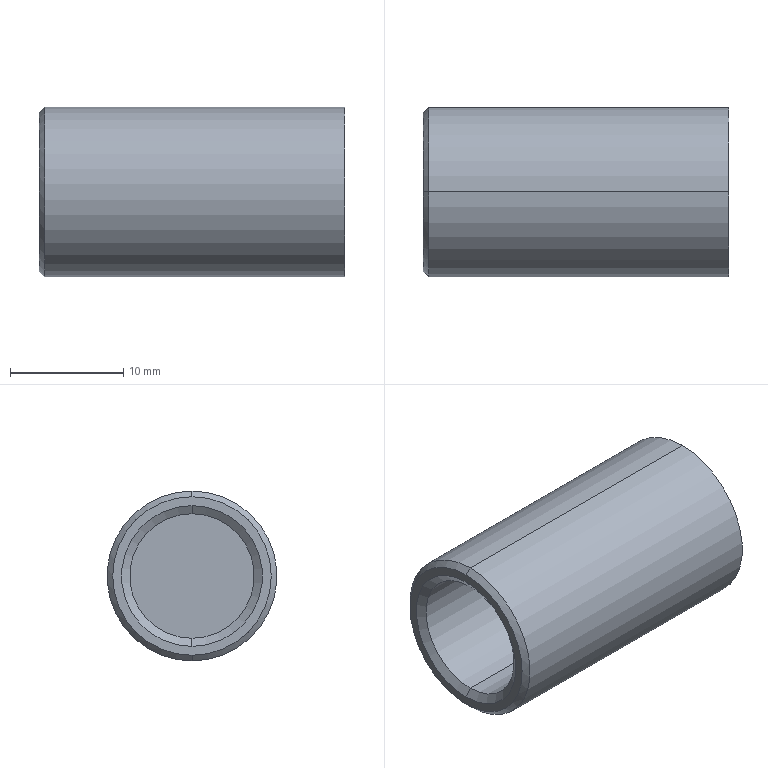Component | SolidWorks | LocatingPin-1 | 1 solid | 11 faces | box 27 x 15 x 15 mm | volume 2953 mm3 | cylinder 4 | cone 4 | plane 3 | commonest cylinder face diameters 11 x2 15 x2 | material Alloy Steel
build123d program:
from build123d import *


with BuildPart() as part:
    # Model → Revolve1 (revolve)
    with BuildSketch(Plane.XY, mode=Mode.PRIVATE) as revolve1_sk:
        Polygon((10.636, 8.083), (-15.864, 8.083), (-16.364, 7.583), (-16.364, 6.802), (-15.864, 6.083), (2.636, 6.083), (2.636, 0.5825), (10.636, 0.5825), align=None)
    revolve(revolve1_sk.sketch.rotate(Axis((10.636, 0.5825, 0), (-1, 0, 0)), 90), axis=Axis((10.636, 0.5825, 0), (-1, 0, 0)))


solid = part.part

# Placed as in the assembly
solid = solid.moved(Location((92.868, -0.6058, -0.0004174), (0, 0, 0)))
STEP:
#1=COLOUR_RGB('',0.7922,0.8196,0.9333);
#2=FILL_AREA_STYLE_COLOUR('',#1);
#3=FILL_AREA_STYLE('',(#2));
#4=SURFACE_STYLE_FILL_AREA(#3);
#5=SURFACE_SIDE_STYLE('',(#4));
#6=SURFACE_STYLE_USAGE(.BOTH.,#5);
#7=PRESENTATION_STYLE_ASSIGNMENT((#6));
#8=CARTESIAN_POINT('',(3.032,-0.0009151,0.2165));
#9=VERTEX_POINT('',#8);
#10=CARTESIAN_POINT('',(3.032,-0.0009151,-0.2166));
#11=VERTEX_POINT('',#10);
#12=CARTESIAN_POINT('',(3.032,-0.0009151,-0.00001643));
#13=DIRECTION('',(1.,0.,0.));
#14=DIRECTION('',(0.,0.,-1.));
#15=AXIS2_PLACEMENT_3D('',#12,#13,#14);
#16=CIRCLE('',#15,0.2165);
#17=EDGE_CURVE('',#9,#11,#16,.T.);
#18=ORIENTED_EDGE('',*,*,#17,.F.);
#19=CARTESIAN_POINT('',(3.76,-0.0009151,0.2165));
#20=VERTEX_POINT('',#19);
#21=CARTESIAN_POINT('',(4.075,-0.0009151,0.2165));
#22=DIRECTION('',(1.,0.,0.));
#23=VECTOR('',#22,39.37);
#24=LINE('',#21,#23);
#25=EDGE_CURVE('',#9,#20,#24,.T.);
#26=ORIENTED_EDGE('',*,*,#25,.T.);
#27=CARTESIAN_POINT('',(3.76,-0.0009151,-0.2166));
#28=VERTEX_POINT('',#27);
#29=CARTESIAN_POINT('',(3.76,-0.0009151,-0.00001643));
#30=DIRECTION('',(1.,0.,0.));
#31=DIRECTION('',(0.,0.,-1.));
#32=AXIS2_PLACEMENT_3D('',#29,#30,#31);
#33=CIRCLE('',#32,0.2165);
#34=EDGE_CURVE('',#20,#28,#33,.T.);
#35=ORIENTED_EDGE('',*,*,#34,.T.);
#36=CARTESIAN_POINT('',(4.075,-0.0009151,-0.2166));
#37=DIRECTION('',(1.,0.,0.));
#38=VECTOR('',#37,39.37);
#39=LINE('',#36,#38);
#40=EDGE_CURVE('',#11,#28,#39,.T.);
#41=ORIENTED_EDGE('',*,*,#40,.F.);
#42=EDGE_LOOP('',(#18,#26,#35,#41));
#43=FACE_OUTER_BOUND('',#42,.T.);
#44=CARTESIAN_POINT('',(4.075,-0.0009151,-0.00001643));
#45=DIRECTION('',(1.,0.,0.));
#46=DIRECTION('',(0.,0.,-1.));
#47=AXIS2_PLACEMENT_3D('',#44,#45,#46);
#48=CYLINDRICAL_SURFACE('',#47,0.2165);
#49=ADVANCED_FACE('',(#43),#48,.F.);
#50=ORIENTED_EDGE('',*,*,#17,.T.);
#51=CARTESIAN_POINT('',(3.012,-0.0009151,-0.2449));
#52=VERTEX_POINT('',#51);
#53=CARTESIAN_POINT('',(3.012,-0.0009151,-0.2449));
#54=DIRECTION('',(-0.5705,0.,-0.8213));
#55=VECTOR('',#54,39.37);
#56=LINE('',#53,#55);
#57=EDGE_CURVE('',#11,#52,#56,.T.);
#58=ORIENTED_EDGE('',*,*,#57,.T.);
#59=CARTESIAN_POINT('',(3.012,-0.0009151,0.2449));
#60=VERTEX_POINT('',#59);
#61=CARTESIAN_POINT('',(3.012,-0.0009151,-0.00001643));
#62=DIRECTION('',(1.,0.,0.));
#63=DIRECTION('',(0.,0.,-1.));
#64=AXIS2_PLACEMENT_3D('',#61,#62,#63);
#65=CIRCLE('',#64,0.2449);
#66=EDGE_CURVE('',#60,#52,#65,.T.);
#67=ORIENTED_EDGE('',*,*,#66,.F.);
#68=CARTESIAN_POINT('',(3.012,-0.0009151,0.2449));
#69=DIRECTION('',(-0.5705,0.,0.8213));
#70=VECTOR('',#69,39.37);
#71=LINE('',#68,#70);
#72=EDGE_CURVE('',#9,#60,#71,.T.);
#73=ORIENTED_EDGE('',*,*,#72,.F.);
#74=EDGE_LOOP('',(#50,#58,#67,#73));
#75=FACE_OUTER_BOUND('',#74,.T.);
#76=CARTESIAN_POINT('',(3.012,-0.0009151,-0.00001643));
#77=DIRECTION('',(-1.,0.,0.));
#78=DIRECTION('',(0.,0.,1.));
#79=AXIS2_PLACEMENT_3D('',#76,#77,#78);
#80=CONICAL_SURFACE('',#79,0.2449,0.9637);
#81=ADVANCED_FACE('',(#75),#80,.F.);
#82=CARTESIAN_POINT('',(3.012,-0.0009151,-0.2756));
#83=VERTEX_POINT('',#82);
#84=CARTESIAN_POINT('',(3.012,-0.0009151,0.2756));
#85=VERTEX_POINT('',#84);
#86=CARTESIAN_POINT('',(3.012,-0.0009151,-0.00001643));
#87=DIRECTION('',(1.,0.,0.));
#88=DIRECTION('',(0.,0.,-1.));
#89=AXIS2_PLACEMENT_3D('',#86,#87,#88);
#90=CIRCLE('',#89,0.2756);
#91=EDGE_CURVE('',#83,#85,#90,.T.);
#92=ORIENTED_EDGE('',*,*,#91,.T.);
#93=CARTESIAN_POINT('',(3.032,-0.0009151,0.2953));
#94=VERTEX_POINT('',#93);
#95=CARTESIAN_POINT('',(3.032,-0.0009151,0.2953));
#96=DIRECTION('',(0.7071,0.,0.7071));
#97=VECTOR('',#96,39.37);
#98=LINE('',#95,#97);
#99=EDGE_CURVE('',#85,#94,#98,.T.);
#100=ORIENTED_EDGE('',*,*,#99,.T.);
#101=CARTESIAN_POINT('',(3.032,-0.0009151,-0.2953));
#102=VERTEX_POINT('',#101);
#103=CARTESIAN_POINT('',(3.032,-0.0009151,-0.00001643));
#104=DIRECTION('',(1.,0.,0.));
#105=DIRECTION('',(0.,0.,-1.));
#106=AXIS2_PLACEMENT_3D('',#103,#104,#105);
#107=CIRCLE('',#106,0.2953);
#108=EDGE_CURVE('',#102,#94,#107,.T.);
#109=ORIENTED_EDGE('',*,*,#108,.F.);
#110=CARTESIAN_POINT('',(3.032,-0.0009151,-0.2953));
#111=DIRECTION('',(0.7071,0.,-0.7071));
#112=VECTOR('',#111,39.37);
#113=LINE('',#110,#112);
#114=EDGE_CURVE('',#83,#102,#113,.T.);
#115=ORIENTED_EDGE('',*,*,#114,.F.);
#116=EDGE_LOOP('',(#92,#100,#109,#115));
#117=FACE_OUTER_BOUND('',#116,.T.);
#118=CARTESIAN_POINT('',(3.032,-0.0009151,-0.00001643));
#119=DIRECTION('',(1.,0.,0.));
#120=DIRECTION('',(0.,0.,-1.));
#121=AXIS2_PLACEMENT_3D('',#118,#119,#120);
#122=CONICAL_SURFACE('',#121,0.2953,0.7854);
#123=ADVANCED_FACE('',(#117),#122,.T.);
#124=ORIENTED_EDGE('',*,*,#108,.T.);
#125=CARTESIAN_POINT('',(4.075,-0.0009151,0.2953));
#126=VERTEX_POINT('',#125);
#127=CARTESIAN_POINT('',(4.075,-0.0009151,0.2953));
#128=DIRECTION('',(1.,0.,0.));
#129=VECTOR('',#128,39.37);
#130=LINE('',#127,#129);
#131=EDGE_CURVE('',#94,#126,#130,.T.);
#132=ORIENTED_EDGE('',*,*,#131,.T.);
#133=CARTESIAN_POINT('',(4.075,-0.0009151,-0.2953));
#134=VERTEX_POINT('',#133);
#135=CARTESIAN_POINT('',(4.075,-0.0009151,-0.00001643));
#136=DIRECTION('',(1.,0.,0.));
#137=DIRECTION('',(0.,0.,-1.));
#138=AXIS2_PLACEMENT_3D('',#135,#136,#137);
#139=CIRCLE('',#138,0.2953);
#140=EDGE_CURVE('',#134,#126,#139,.T.);
#141=ORIENTED_EDGE('',*,*,#140,.F.);
#142=CARTESIAN_POINT('',(4.075,-0.0009151,-0.2953));
#143=DIRECTION('',(1.,0.,0.));
#144=VECTOR('',#143,39.37);
#145=LINE('',#142,#144);
#146=EDGE_CURVE('',#102,#134,#145,.T.);
#147=ORIENTED_EDGE('',*,*,#146,.F.);
#148=EDGE_LOOP('',(#124,#132,#141,#147));
#149=FACE_OUTER_BOUND('',#148,.T.);
#150=CARTESIAN_POINT('',(4.075,-0.0009151,-0.00001643));
#151=DIRECTION('',(1.,0.,0.));
#152=DIRECTION('',(0.,0.,-1.));
#153=AXIS2_PLACEMENT_3D('',#150,#151,#152);
#154=CYLINDRICAL_SURFACE('',#153,0.2953);
#155=ADVANCED_FACE('',(#149),#154,.T.);
#156=ORIENTED_EDGE('',*,*,#140,.T.);
#157=CARTESIAN_POINT('',(4.075,-0.0009151,-0.00001643));
#158=DIRECTION('',(1.,0.,0.));
#159=DIRECTION('',(0.,0.,-1.));
#160=AXIS2_PLACEMENT_3D('',#157,#158,#159);
#161=CIRCLE('',#160,0.2953);
#162=EDGE_CURVE('',#126,#134,#161,.T.);
#163=ORIENTED_EDGE('',*,*,#162,.T.);
#164=EDGE_LOOP('',(#156,#163));
#165=FACE_OUTER_BOUND('',#164,.T.);
#166=CARTESIAN_POINT('',(4.075,-0.0009151,-0.00001643));
#167=DIRECTION('',(1.,0.,0.));
#168=DIRECTION('',(0.,0.,-1.));
#169=AXIS2_PLACEMENT_3D('',#166,#167,#168);
#170=PLANE('',#169);
#171=ADVANCED_FACE('',(#165),#170,.T.);
#172=ORIENTED_EDGE('',*,*,#131,.F.);
#173=CARTESIAN_POINT('',(3.032,-0.0009151,-0.00001643));
#174=DIRECTION('',(1.,0.,0.));
#175=DIRECTION('',(0.,0.,-1.));
#176=AXIS2_PLACEMENT_3D('',#173,#174,#175);
#177=CIRCLE('',#176,0.2953);
#178=EDGE_CURVE('',#94,#102,#177,.T.);
#179=ORIENTED_EDGE('',*,*,#178,.T.);
#180=ORIENTED_EDGE('',*,*,#146,.T.);
#181=ORIENTED_EDGE('',*,*,#162,.F.);
#182=EDGE_LOOP('',(#172,#179,#180,#181));
#183=FACE_OUTER_BOUND('',#182,.T.);
#184=CARTESIAN_POINT('',(4.075,-0.0009151,-0.00001643));
#185=DIRECTION('',(1.,0.,0.));
#186=DIRECTION('',(0.,0.,-1.));
#187=AXIS2_PLACEMENT_3D('',#184,#185,#186);
#188=CYLINDRICAL_SURFACE('',#187,0.2953);
#189=ADVANCED_FACE('',(#183),#188,.T.);
#190=ORIENTED_EDGE('',*,*,#99,.F.);
#191=CARTESIAN_POINT('',(3.012,-0.0009151,-0.00001643));
#192=DIRECTION('',(1.,0.,0.));
#193=DIRECTION('',(0.,0.,-1.));
#194=AXIS2_PLACEMENT_3D('',#191,#192,#193);
#195=CIRCLE('',#194,0.2756);
#196=EDGE_CURVE('',#85,#83,#195,.T.);
#197=ORIENTED_EDGE('',*,*,#196,.T.);
#198=ORIENTED_EDGE('',*,*,#114,.T.);
#199=ORIENTED_EDGE('',*,*,#178,.F.);
#200=EDGE_LOOP('',(#190,#197,#198,#199));
#201=FACE_OUTER_BOUND('',#200,.T.);
#202=CARTESIAN_POINT('',(3.032,-0.0009151,-0.00001643));
#203=DIRECTION('',(1.,0.,0.));
#204=DIRECTION('',(0.,0.,-1.));
#205=AXIS2_PLACEMENT_3D('',#202,#203,#204);
#206=CONICAL_SURFACE('',#205,0.2953,0.7854);
#207=ADVANCED_FACE('',(#201),#206,.T.);
#208=ORIENTED_EDGE('',*,*,#66,.T.);
#209=CARTESIAN_POINT('',(3.012,-0.0009151,-0.00001643));
#210=DIRECTION('',(1.,0.,0.));
#211=DIRECTION('',(0.,0.,-1.));
#212=AXIS2_PLACEMENT_3D('',#209,#210,#211);
#213=CIRCLE('',#212,0.2449);
#214=EDGE_CURVE('',#52,#60,#213,.T.);
#215=ORIENTED_EDGE('',*,*,#214,.T.);
#216=EDGE_LOOP('',(#208,#215));
#217=FACE_BOUND('',#216,.T.);
#218=ORIENTED_EDGE('',*,*,#91,.F.);
#219=ORIENTED_EDGE('',*,*,#196,.F.);
#220=EDGE_LOOP('',(#218,#219));
#221=FACE_OUTER_BOUND('',#220,.T.);
#222=CARTESIAN_POINT('',(3.012,0.244,-0.00001643));
#223=DIRECTION('',(-1.,0.,0.));
#224=DIRECTION('',(0.,0.,1.));
#225=AXIS2_PLACEMENT_3D('',#222,#223,#224);
#226=PLANE('',#225);
#227=ADVANCED_FACE('',(#217,#221),#226,.T.);
#228=ORIENTED_EDGE('',*,*,#57,.F.);
#229=CARTESIAN_POINT('',(3.032,-0.0009151,-0.00001643));
#230=DIRECTION('',(1.,0.,0.));
#231=DIRECTION('',(0.,0.,-1.));
#232=AXIS2_PLACEMENT_3D('',#229,#230,#231);
#233=CIRCLE('',#232,0.2165);
#234=EDGE_CURVE('',#11,#9,#233,.T.);
#235=ORIENTED_EDGE('',*,*,#234,.T.);
#236=ORIENTED_EDGE('',*,*,#72,.T.);
#237=ORIENTED_EDGE('',*,*,#214,.F.);
#238=EDGE_LOOP('',(#228,#235,#236,#237));
#239=FACE_OUTER_BOUND('',#238,.T.);
#240=CARTESIAN_POINT('',(3.012,-0.0009151,-0.00001643));
#241=DIRECTION('',(-1.,0.,0.));
#242=DIRECTION('',(0.,0.,1.));
#243=AXIS2_PLACEMENT_3D('',#240,#241,#242);
#244=CONICAL_SURFACE('',#243,0.2449,0.9637);
#245=ADVANCED_FACE('',(#239),#244,.F.);
#246=ORIENTED_EDGE('',*,*,#25,.F.);
#247=ORIENTED_EDGE('',*,*,#234,.F.);
#248=ORIENTED_EDGE('',*,*,#40,.T.);
#249=CARTESIAN_POINT('',(3.76,-0.0009151,-0.00001643));
#250=DIRECTION('',(1.,0.,0.));
#251=DIRECTION('',(0.,0.,-1.));
#252=AXIS2_PLACEMENT_3D('',#249,#250,#251);
#253=CIRCLE('',#252,0.2165);
#254=EDGE_CURVE('',#28,#20,#253,.T.);
#255=ORIENTED_EDGE('',*,*,#254,.T.);
#256=EDGE_LOOP('',(#246,#247,#248,#255));
#257=FACE_OUTER_BOUND('',#256,.T.);
#258=CARTESIAN_POINT('',(4.075,-0.0009151,-0.00001643));
#259=DIRECTION('',(1.,0.,0.));
#260=DIRECTION('',(0.,0.,-1.));
#261=AXIS2_PLACEMENT_3D('',#258,#259,#260);
#262=CYLINDRICAL_SURFACE('',#261,0.2165);
#263=ADVANCED_FACE('',(#257),#262,.F.);
#264=ORIENTED_EDGE('',*,*,#254,.F.);
#265=ORIENTED_EDGE('',*,*,#34,.F.);
#266=EDGE_LOOP('',(#264,#265));
#267=FACE_OUTER_BOUND('',#266,.T.);
#268=CARTESIAN_POINT('',(3.76,-0.0009151,-0.00001643));
#269=DIRECTION('',(-1.,0.,0.));
#270=DIRECTION('',(0.,0.,1.));
#271=AXIS2_PLACEMENT_3D('',#268,#269,#270);
#272=PLANE('',#271);
#273=ADVANCED_FACE('',(#267),#272,.T.);
#274=CLOSED_SHELL('',(#49,#81,#123,#155,#171,#189,#207,#227,#245,#263,#273));
#275=MANIFOLD_SOLID_BREP('',#274);
#276=STYLED_ITEM('',(#7),#275);
#277=PRESENTATION_LAYER_ASSIGNMENT('','',(#276));
#278=CARTESIAN_POINT('',(0.,0.,0.));
#279=DIRECTION('',(0.,0.,1.));
#280=DIRECTION('',(1.,0.,0.));
#281=AXIS2_PLACEMENT_3D('',#278,#279,#280);
#282=(LENGTH_UNIT()NAMED_UNIT(*)SI_UNIT($,.METRE.));
#283=LENGTH_MEASURE_WITH_UNIT(LENGTH_MEASURE(0.0254),#282);
#284=DIMENSIONAL_EXPONENTS(1.,0.,0.,0.,0.,0.,0.);
#285=(CONVERSION_BASED_UNIT('',#283)LENGTH_UNIT()NAMED_UNIT(#284));
#286=UNCERTAINTY_MEASURE_WITH_UNIT(LENGTH_MEASURE(0.00001),#285,'','');
#287=(NAMED_UNIT(*)PLANE_ANGLE_UNIT()SI_UNIT($,.RADIAN.));
#288=(NAMED_UNIT(*)SI_UNIT($,.STERADIAN.)SOLID_ANGLE_UNIT());
#289=(GEOMETRIC_REPRESENTATION_CONTEXT(3)GLOBAL_UNCERTAINTY_ASSIGNED_CONTEXT((#286))GLOBAL_UNIT_ASSIGNED_CONTEXT((#285,#287,#288))REPRESENTATION_CONTEXT('',''));
#290=ADVANCED_BREP_SHAPE_REPRESENTATION('',(#275,#281),#289);
#291=(LENGTH_UNIT()NAMED_UNIT(*)SI_UNIT($,.METRE.));
#292=LENGTH_MEASURE_WITH_UNIT(LENGTH_MEASURE(0.0254),#291);
#293=DIMENSIONAL_EXPONENTS(1.,0.,0.,0.,0.,0.,0.);
#294=(CONVERSION_BASED_UNIT('',#292)LENGTH_UNIT()NAMED_UNIT(#293));
#295=UNCERTAINTY_MEASURE_WITH_UNIT(LENGTH_MEASURE(0.00001),#294,'','');
#296=(NAMED_UNIT(*)PLANE_ANGLE_UNIT()SI_UNIT($,.RADIAN.));
#297=(NAMED_UNIT(*)SI_UNIT($,.STERADIAN.)SOLID_ANGLE_UNIT());
#298=(GEOMETRIC_REPRESENTATION_CONTEXT(3)GLOBAL_UNCERTAINTY_ASSIGNED_CONTEXT((#295))GLOBAL_UNIT_ASSIGNED_CONTEXT((#294,#296,#297))REPRESENTATION_CONTEXT('',''));
#299=MECHANICAL_DESIGN_GEOMETRIC_PRESENTATION_REPRESENTATION('',(#276),#298);